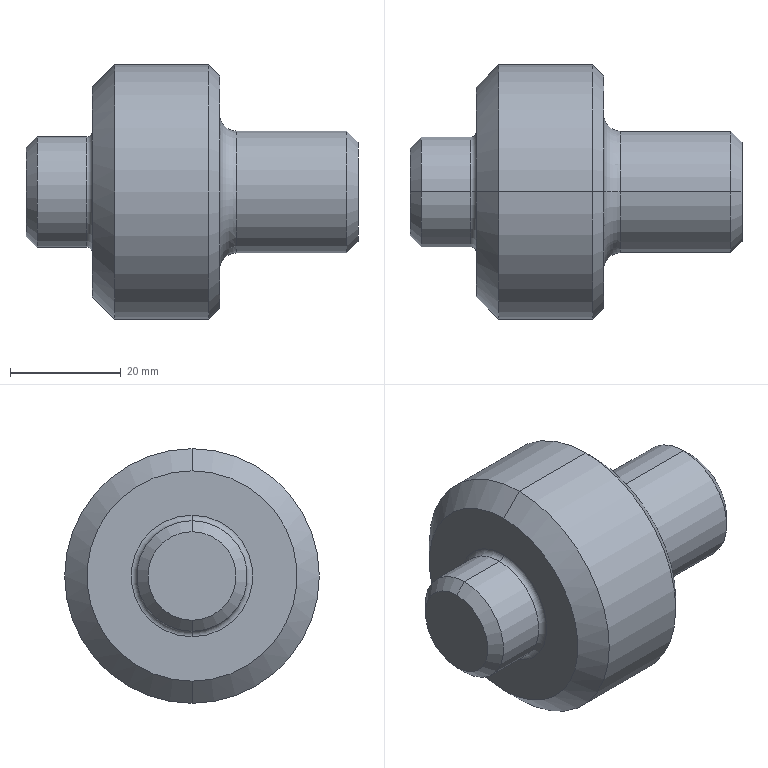Component | SolidWorks | THK-A1028TravelingMotorFlangeMountingAxis-1 | 1 solid | 26 faces | box 60 x 46 x 46 mm | volume 48569 mm3 | cone 10 | cylinder 8 | torus 4 | plane 4 | commonest cylinder face diameters 8.5 x2 22 x2 46 x2 20 x2 | material 45
build123d program:
from build123d import *

# Parameters (mm, degrees)
SKETCH1_R              = 10
BOSS_EXTRUDE1_DEPTH    = 6
SKETCH2_R              = 23
BOSS_EXTRUDE2_DEPTH    = 23
SKETCH3_R              = 11
BOSS_EXTRUDE3_DEPTH    = 25
M10_TAPPED_HOLE1_D     = 8.5
M10_TAPPED_HOLE1_DEPTH = 25
M10_TAPPED_HOLE1_TIP   = 2.554
CHAMFER1_SIZE          = 2
FILLET1_R              = 3
FILLET2_R              = 1
CHAMFER2_SIZE          = 4


with BuildPart() as part:
    # Sketch1 → Boss-Extrude1 (new, symmetric)
    with BuildSketch(Plane(origin=(0, 0, 0), x_dir=(0, 0, -1), z_dir=(1, 0, 0))):
        Circle(SKETCH1_R)
    extrude(amount=BOSS_EXTRUDE1_DEPTH, both=True)

    # Sketch2 → Boss-Extrude2 (add)
    with BuildSketch(Plane.ZY.offset(-6)):
        Circle(SKETCH2_R)
    extrude(amount=-BOSS_EXTRUDE2_DEPTH)

    # Sketch3 → Boss-Extrude3 (add)
    with BuildSketch(Plane.ZY.offset(-29)):
        Circle(SKETCH3_R)
    extrude(amount=-BOSS_EXTRUDE3_DEPTH)

    # M10 Tapped Hole1
    with Locations(Plane(origin=(54, 0, 0), x_dir=(0, 0, -1), z_dir=(1, 0, 0))):
        with Locations((0, 0)):
            Hole(M10_TAPPED_HOLE1_D / 2, depth=M10_TAPPED_HOLE1_DEPTH)
            with Locations((0, 0, -(M10_TAPPED_HOLE1_DEPTH + M10_TAPPED_HOLE1_TIP / 2))):  # 118° drill point
                Cone(0, M10_TAPPED_HOLE1_D / 2, M10_TAPPED_HOLE1_TIP, mode=Mode.SUBTRACT)

    # Chamfer1
    chamfer1_edges = [part.edges().sort_by_distance(p)[0] for p in [
        (54, 0, -11),
        (-6, 0, 10),
        (29, 0, -23),
    ]]
    chamfer(chamfer1_edges, length=CHAMFER1_SIZE)

    # Fillet1
    fillet1_edges = [part.edges().sort_by_distance(p)[0] for p in [
        (29, 0, -11),
    ]]
    fillet(fillet1_edges, radius=FILLET1_R)

    # Fillet2
    fillet2_edges = [part.edges().sort_by_distance(p)[0] for p in [
        (6, 0, 10),
    ]]
    fillet(fillet2_edges, radius=FILLET2_R)

    # Chamfer2
    chamfer2_edges = [part.edges().sort_by_distance(p)[0] for p in [
        (6, 0, -23),
    ]]
    chamfer(chamfer2_edges, length=CHAMFER2_SIZE)


solid = part.part

# Placed as in the assembly
solid = solid.moved(Location((79, 115, 321), (0, 0, 0)))
STEP:
#1=CARTESIAN_POINT('',(3.346,4.528,13.386));
#2=VERTEX_POINT('',#1);
#3=CARTESIAN_POINT('',(3.346,4.528,11.89));
#4=VERTEX_POINT('',#3);
#5=CARTESIAN_POINT('',(3.346,4.528,12.638));
#6=DIRECTION('',(-1.,0.,-0.));
#7=DIRECTION('',(0.,0.,1.));
#8=AXIS2_PLACEMENT_3D('',#5,#6,#7);
#9=CIRCLE('',#8,0.748);
#10=EDGE_CURVE('',#2,#4,#9,.T.);
#11=ORIENTED_EDGE('',*,*,#10,.F.);
#12=CARTESIAN_POINT('',(3.504,4.528,13.543));
#13=VERTEX_POINT('',#12);
#14=CARTESIAN_POINT('',(3.346,4.528,13.386));
#15=DIRECTION('',(0.7071,0.,0.7071));
#16=VECTOR('',#15,39.37);
#17=LINE('',#14,#16);
#18=EDGE_CURVE('',#2,#13,#17,.T.);
#19=ORIENTED_EDGE('',*,*,#18,.T.);
#20=CARTESIAN_POINT('',(3.504,4.528,11.732));
#21=VERTEX_POINT('',#20);
#22=CARTESIAN_POINT('',(3.504,4.528,12.638));
#23=DIRECTION('',(1.,0.,0.));
#24=DIRECTION('',(0.,0.,1.));
#25=AXIS2_PLACEMENT_3D('',#22,#23,#24);
#26=CIRCLE('',#25,0.9055);
#27=EDGE_CURVE('',#21,#13,#26,.T.);
#28=ORIENTED_EDGE('',*,*,#27,.F.);
#29=CARTESIAN_POINT('',(3.346,4.528,11.89));
#30=DIRECTION('',(0.7071,0.,-0.7071));
#31=VECTOR('',#30,39.37);
#32=LINE('',#29,#31);
#33=EDGE_CURVE('',#4,#21,#32,.T.);
#34=ORIENTED_EDGE('',*,*,#33,.F.);
#35=EDGE_LOOP('',(#11,#19,#28,#34));
#36=FACE_OUTER_BOUND('',#35,.T.);
#37=CARTESIAN_POINT('',(3.346,4.528,12.638));
#38=DIRECTION('',(1.,0.,0.));
#39=DIRECTION('',(0.,0.,-1.));
#40=AXIS2_PLACEMENT_3D('',#37,#38,#39);
#41=CONICAL_SURFACE('',#40,0.748,0.7854);
#42=ADVANCED_FACE('',(#36),#41,.T.);
#43=CARTESIAN_POINT('',(3.307,4.528,12.244));
#44=VERTEX_POINT('',#43);
#45=CARTESIAN_POINT('',(3.307,4.528,13.031));
#46=VERTEX_POINT('',#45);
#47=CARTESIAN_POINT('',(3.307,4.528,12.638));
#48=DIRECTION('',(-1.,0.,-0.));
#49=DIRECTION('',(0.,0.,1.));
#50=AXIS2_PLACEMENT_3D('',#47,#48,#49);
#51=CIRCLE('',#50,0.3937);
#52=EDGE_CURVE('',#44,#46,#51,.T.);
#53=ORIENTED_EDGE('',*,*,#52,.F.);
#54=CARTESIAN_POINT('',(3.346,4.528,12.205));
#55=VERTEX_POINT('',#54);
#56=CARTESIAN_POINT('',(3.307,4.528,12.205));
#57=DIRECTION('',(-0.,1.,0.));
#58=DIRECTION('',(0.,0.,1.));
#59=AXIS2_PLACEMENT_3D('',#56,#57,#58);
#60=CIRCLE('',#59,0.03937);
#61=EDGE_CURVE('',#44,#55,#60,.T.);
#62=ORIENTED_EDGE('',*,*,#61,.T.);
#63=CARTESIAN_POINT('',(3.346,4.528,13.071));
#64=VERTEX_POINT('',#63);
#65=CARTESIAN_POINT('',(3.346,4.528,12.638));
#66=DIRECTION('',(1.,0.,0.));
#67=DIRECTION('',(0.,0.,1.));
#68=AXIS2_PLACEMENT_3D('',#65,#66,#67);
#69=CIRCLE('',#68,0.4331);
#70=EDGE_CURVE('',#64,#55,#69,.T.);
#71=ORIENTED_EDGE('',*,*,#70,.F.);
#72=CARTESIAN_POINT('',(3.307,4.528,13.071));
#73=DIRECTION('',(0.,-1.,0.));
#74=DIRECTION('',(0.,0.,-1.));
#75=AXIS2_PLACEMENT_3D('',#72,#73,#74);
#76=CIRCLE('',#75,0.03937);
#77=EDGE_CURVE('',#46,#64,#76,.T.);
#78=ORIENTED_EDGE('',*,*,#77,.F.);
#79=EDGE_LOOP('',(#53,#62,#71,#78));
#80=FACE_OUTER_BOUND('',#79,.T.);
#81=CARTESIAN_POINT('',(3.307,4.528,12.638));
#82=DIRECTION('',(-1.,0.,-0.));
#83=DIRECTION('',(-0.,0.,1.));
#84=AXIS2_PLACEMENT_3D('',#81,#82,#83);
#85=TOROIDAL_SURFACE('',#84,0.4331,0.03937);
#86=ADVANCED_FACE('',(#80),#85,.F.);
#87=CARTESIAN_POINT('',(4.252,4.528,12.087));
#88=VERTEX_POINT('',#87);
#89=CARTESIAN_POINT('',(4.252,4.528,13.189));
#90=VERTEX_POINT('',#89);
#91=CARTESIAN_POINT('',(4.252,4.528,12.638));
#92=DIRECTION('',(-1.,0.,-0.));
#93=DIRECTION('',(0.,0.,1.));
#94=AXIS2_PLACEMENT_3D('',#91,#92,#93);
#95=CIRCLE('',#94,0.5512);
#96=EDGE_CURVE('',#88,#90,#95,.T.);
#97=ORIENTED_EDGE('',*,*,#96,.F.);
#98=CARTESIAN_POINT('',(4.37,4.528,12.205));
#99=VERTEX_POINT('',#98);
#100=CARTESIAN_POINT('',(4.37,4.528,12.087));
#101=DIRECTION('',(-0.,1.,0.));
#102=DIRECTION('',(0.,0.,1.));
#103=AXIS2_PLACEMENT_3D('',#100,#101,#102);
#104=CIRCLE('',#103,0.1181);
#105=EDGE_CURVE('',#88,#99,#104,.T.);
#106=ORIENTED_EDGE('',*,*,#105,.T.);
#107=CARTESIAN_POINT('',(4.37,4.528,13.071));
#108=VERTEX_POINT('',#107);
#109=CARTESIAN_POINT('',(4.37,4.528,12.638));
#110=DIRECTION('',(1.,0.,0.));
#111=DIRECTION('',(0.,0.,1.));
#112=AXIS2_PLACEMENT_3D('',#109,#110,#111);
#113=CIRCLE('',#112,0.4331);
#114=EDGE_CURVE('',#108,#99,#113,.T.);
#115=ORIENTED_EDGE('',*,*,#114,.F.);
#116=CARTESIAN_POINT('',(4.37,4.528,13.189));
#117=DIRECTION('',(0.,-1.,0.));
#118=DIRECTION('',(0.,0.,-1.));
#119=AXIS2_PLACEMENT_3D('',#116,#117,#118);
#120=CIRCLE('',#119,0.1181);
#121=EDGE_CURVE('',#90,#108,#120,.T.);
#122=ORIENTED_EDGE('',*,*,#121,.F.);
#123=EDGE_LOOP('',(#97,#106,#115,#122));
#124=FACE_OUTER_BOUND('',#123,.T.);
#125=CARTESIAN_POINT('',(4.37,4.528,12.638));
#126=DIRECTION('',(-1.,0.,-0.));
#127=DIRECTION('',(-0.,0.,1.));
#128=AXIS2_PLACEMENT_3D('',#125,#126,#127);
#129=TOROIDAL_SURFACE('',#128,0.5512,0.1181);
#130=ADVANCED_FACE('',(#124),#129,.F.);
#131=CARTESIAN_POINT('',(4.252,4.528,11.811));
#132=VERTEX_POINT('',#131);
#133=CARTESIAN_POINT('',(4.252,4.528,13.465));
#134=VERTEX_POINT('',#133);
#135=CARTESIAN_POINT('',(4.252,4.528,12.638));
#136=DIRECTION('',(1.,0.,0.));
#137=DIRECTION('',(0.,0.,1.));
#138=AXIS2_PLACEMENT_3D('',#135,#136,#137);
#139=CIRCLE('',#138,0.8268);
#140=EDGE_CURVE('',#132,#134,#139,.T.);
#141=ORIENTED_EDGE('',*,*,#140,.F.);
#142=CARTESIAN_POINT('',(4.173,4.528,11.732));
#143=VERTEX_POINT('',#142);
#144=CARTESIAN_POINT('',(4.173,4.528,11.732));
#145=DIRECTION('',(-0.7071,0.,-0.7071));
#146=VECTOR('',#145,39.37);
#147=LINE('',#144,#146);
#148=EDGE_CURVE('',#132,#143,#147,.T.);
#149=ORIENTED_EDGE('',*,*,#148,.T.);
#150=CARTESIAN_POINT('',(4.173,4.528,13.543));
#151=VERTEX_POINT('',#150);
#152=CARTESIAN_POINT('',(4.173,4.528,12.638));
#153=DIRECTION('',(-1.,0.,-0.));
#154=DIRECTION('',(0.,0.,1.));
#155=AXIS2_PLACEMENT_3D('',#152,#153,#154);
#156=CIRCLE('',#155,0.9055);
#157=EDGE_CURVE('',#151,#143,#156,.T.);
#158=ORIENTED_EDGE('',*,*,#157,.F.);
#159=CARTESIAN_POINT('',(4.173,4.528,13.543));
#160=DIRECTION('',(-0.7071,0.,0.7071));
#161=VECTOR('',#160,39.37);
#162=LINE('',#159,#161);
#163=EDGE_CURVE('',#134,#151,#162,.T.);
#164=ORIENTED_EDGE('',*,*,#163,.F.);
#165=EDGE_LOOP('',(#141,#149,#158,#164));
#166=FACE_OUTER_BOUND('',#165,.T.);
#167=CARTESIAN_POINT('',(4.173,4.528,12.638));
#168=DIRECTION('',(-1.,0.,-0.));
#169=DIRECTION('',(0.,0.,1.));
#170=AXIS2_PLACEMENT_3D('',#167,#168,#169);
#171=CONICAL_SURFACE('',#170,0.9055,0.7854);
#172=ADVANCED_FACE('',(#166),#171,.T.);
#173=CARTESIAN_POINT('',(5.236,4.528,12.283));
#174=VERTEX_POINT('',#173);
#175=CARTESIAN_POINT('',(5.236,4.528,12.992));
#176=VERTEX_POINT('',#175);
#177=CARTESIAN_POINT('',(5.236,4.528,12.638));
#178=DIRECTION('',(1.,0.,0.));
#179=DIRECTION('',(0.,0.,1.));
#180=AXIS2_PLACEMENT_3D('',#177,#178,#179);
#181=CIRCLE('',#180,0.3543);
#182=EDGE_CURVE('',#174,#176,#181,.T.);
#183=ORIENTED_EDGE('',*,*,#182,.F.);
#184=CARTESIAN_POINT('',(5.157,4.528,12.205));
#185=VERTEX_POINT('',#184);
#186=CARTESIAN_POINT('',(5.157,4.528,12.205));
#187=DIRECTION('',(-0.7071,0.,-0.7071));
#188=VECTOR('',#187,39.37);
#189=LINE('',#186,#188);
#190=EDGE_CURVE('',#174,#185,#189,.T.);
#191=ORIENTED_EDGE('',*,*,#190,.T.);
#192=CARTESIAN_POINT('',(5.157,4.528,13.071));
#193=VERTEX_POINT('',#192);
#194=CARTESIAN_POINT('',(5.157,4.528,12.638));
#195=DIRECTION('',(-1.,0.,-0.));
#196=DIRECTION('',(0.,0.,1.));
#197=AXIS2_PLACEMENT_3D('',#194,#195,#196);
#198=CIRCLE('',#197,0.4331);
#199=EDGE_CURVE('',#193,#185,#198,.T.);
#200=ORIENTED_EDGE('',*,*,#199,.F.);
#201=CARTESIAN_POINT('',(5.157,4.528,13.071));
#202=DIRECTION('',(-0.7071,0.,0.7071));
#203=VECTOR('',#202,39.37);
#204=LINE('',#201,#203);
#205=EDGE_CURVE('',#176,#193,#204,.T.);
#206=ORIENTED_EDGE('',*,*,#205,.F.);
#207=EDGE_LOOP('',(#183,#191,#200,#206));
#208=FACE_OUTER_BOUND('',#207,.T.);
#209=CARTESIAN_POINT('',(5.157,4.528,12.638));
#210=DIRECTION('',(-1.,0.,-0.));
#211=DIRECTION('',(0.,0.,1.));
#212=AXIS2_PLACEMENT_3D('',#209,#210,#211);
#213=CONICAL_SURFACE('',#212,0.4331,0.7854);
#214=ADVANCED_FACE('',(#208),#213,.T.);
#215=CARTESIAN_POINT('',(2.874,4.528,12.953));
#216=VERTEX_POINT('',#215);
#217=CARTESIAN_POINT('',(2.874,4.528,12.323));
#218=VERTEX_POINT('',#217);
#219=CARTESIAN_POINT('',(2.874,4.528,12.638));
#220=DIRECTION('',(-1.,0.,0.));
#221=DIRECTION('',(0.,0.,-1.));
#222=AXIS2_PLACEMENT_3D('',#219,#220,#221);
#223=CIRCLE('',#222,0.315);
#224=EDGE_CURVE('',#216,#218,#223,.T.);
#225=ORIENTED_EDGE('',*,*,#224,.F.);
#226=CARTESIAN_POINT('',(2.953,4.528,13.031));
#227=VERTEX_POINT('',#226);
#228=CARTESIAN_POINT('',(2.953,4.528,13.031));
#229=DIRECTION('',(0.7071,0.,0.7071));
#230=VECTOR('',#229,39.37);
#231=LINE('',#228,#230);
#232=EDGE_CURVE('',#216,#227,#231,.T.);
#233=ORIENTED_EDGE('',*,*,#232,.T.);
#234=CARTESIAN_POINT('',(2.953,4.528,12.244));
#235=VERTEX_POINT('',#234);
#236=CARTESIAN_POINT('',(2.953,4.528,12.638));
#237=DIRECTION('',(1.,0.,0.));
#238=DIRECTION('',(0.,0.,-1.));
#239=AXIS2_PLACEMENT_3D('',#236,#237,#238);
#240=CIRCLE('',#239,0.3937);
#241=EDGE_CURVE('',#235,#227,#240,.T.);
#242=ORIENTED_EDGE('',*,*,#241,.F.);
#243=CARTESIAN_POINT('',(2.953,4.528,12.244));
#244=DIRECTION('',(0.7071,0.,-0.7071));
#245=VECTOR('',#244,39.37);
#246=LINE('',#243,#245);
#247=EDGE_CURVE('',#218,#235,#246,.T.);
#248=ORIENTED_EDGE('',*,*,#247,.F.);
#249=EDGE_LOOP('',(#225,#233,#242,#248));
#250=FACE_OUTER_BOUND('',#249,.T.);
#251=CARTESIAN_POINT('',(2.953,4.528,12.638));
#252=DIRECTION('',(1.,0.,0.));
#253=DIRECTION('',(0.,0.,-1.));
#254=AXIS2_PLACEMENT_3D('',#251,#252,#253);
#255=CONICAL_SURFACE('',#254,0.3937,0.7854);
#256=ADVANCED_FACE('',(#250),#255,.T.);
#257=CARTESIAN_POINT('',(4.252,4.528,12.805));
#258=VERTEX_POINT('',#257);
#259=CARTESIAN_POINT('',(4.252,4.528,12.47));
#260=VERTEX_POINT('',#259);
#261=CARTESIAN_POINT('',(4.252,4.528,12.638));
#262=DIRECTION('',(1.,0.,0.));
#263=DIRECTION('',(0.,0.,-1.));
#264=AXIS2_PLACEMENT_3D('',#261,#262,#263);
#265=CIRCLE('',#264,0.1673);
#266=EDGE_CURVE('',#258,#260,#265,.T.);
#267=ORIENTED_EDGE('',*,*,#266,.F.);
#268=CARTESIAN_POINT('',(5.236,4.528,12.805));
#269=VERTEX_POINT('',#268);
#270=CARTESIAN_POINT('',(5.236,4.528,12.805));
#271=DIRECTION('',(1.,0.,0.));
#272=VECTOR('',#271,39.37);
#273=LINE('',#270,#272);
#274=EDGE_CURVE('',#258,#269,#273,.T.);
#275=ORIENTED_EDGE('',*,*,#274,.T.);
#276=CARTESIAN_POINT('',(5.236,4.528,12.47));
#277=VERTEX_POINT('',#276);
#278=CARTESIAN_POINT('',(5.236,4.528,12.638));
#279=DIRECTION('',(1.,0.,0.));
#280=DIRECTION('',(0.,0.,-1.));
#281=AXIS2_PLACEMENT_3D('',#278,#279,#280);
#282=CIRCLE('',#281,0.1673);
#283=EDGE_CURVE('',#269,#277,#282,.T.);
#284=ORIENTED_EDGE('',*,*,#283,.T.);
#285=CARTESIAN_POINT('',(5.236,4.528,12.47));
#286=DIRECTION('',(1.,0.,0.));
#287=VECTOR('',#286,39.37);
#288=LINE('',#285,#287);
#289=EDGE_CURVE('',#260,#277,#288,.T.);
#290=ORIENTED_EDGE('',*,*,#289,.F.);
#291=EDGE_LOOP('',(#267,#275,#284,#290));
#292=FACE_OUTER_BOUND('',#291,.T.);
#293=CARTESIAN_POINT('',(5.236,4.528,12.638));
#294=DIRECTION('',(1.,0.,0.));
#295=DIRECTION('',(0.,0.,-1.));
#296=AXIS2_PLACEMENT_3D('',#293,#294,#295);
#297=CYLINDRICAL_SURFACE('',#296,0.1673);
#298=ADVANCED_FACE('',(#292),#297,.F.);
#299=CARTESIAN_POINT('',(4.151,4.528,12.638));
#300=VERTEX_POINT('',#299);
#301=CARTESIAN_POINT('',(4.252,4.528,12.47));
#302=DIRECTION('',(0.515,0.,-0.8572));
#303=VECTOR('',#302,39.37);
#304=LINE('',#301,#303);
#305=EDGE_CURVE('',#300,#260,#304,.T.);
#306=ORIENTED_EDGE('',*,*,#305,.F.);
#307=CARTESIAN_POINT('',(4.252,4.528,12.805));
#308=DIRECTION('',(0.515,0.,0.8572));
#309=VECTOR('',#308,39.37);
#310=LINE('',#307,#309);
#311=EDGE_CURVE('',#300,#258,#310,.T.);
#312=ORIENTED_EDGE('',*,*,#311,.T.);
#313=ORIENTED_EDGE('',*,*,#266,.T.);
#314=EDGE_LOOP('',(#306,#312,#313));
#315=FACE_OUTER_BOUND('',#314,.T.);
#316=CARTESIAN_POINT('',(4.252,4.528,12.638));
#317=DIRECTION('',(1.,0.,0.));
#318=DIRECTION('',(0.,0.,-1.));
#319=AXIS2_PLACEMENT_3D('',#316,#317,#318);
#320=CONICAL_SURFACE('',#319,0.1673,1.03);
#321=ADVANCED_FACE('',(#315),#320,.F.);
#322=ORIENTED_EDGE('',*,*,#199,.T.);
#323=CARTESIAN_POINT('',(5.236,4.528,12.205));
#324=DIRECTION('',(-1.,0.,-0.));
#325=VECTOR('',#324,39.37);
#326=LINE('',#323,#325);
#327=EDGE_CURVE('',#185,#99,#326,.T.);
#328=ORIENTED_EDGE('',*,*,#327,.T.);
#329=CARTESIAN_POINT('',(4.37,4.528,12.638));
#330=DIRECTION('',(1.,0.,0.));
#331=DIRECTION('',(0.,0.,1.));
#332=AXIS2_PLACEMENT_3D('',#329,#330,#331);
#333=CIRCLE('',#332,0.4331);
#334=EDGE_CURVE('',#99,#108,#333,.T.);
#335=ORIENTED_EDGE('',*,*,#334,.T.);
#336=CARTESIAN_POINT('',(5.236,4.528,13.071));
#337=DIRECTION('',(-1.,0.,-0.));
#338=VECTOR('',#337,39.37);
#339=LINE('',#336,#338);
#340=EDGE_CURVE('',#193,#108,#339,.T.);
#341=ORIENTED_EDGE('',*,*,#340,.F.);
#342=EDGE_LOOP('',(#322,#328,#335,#341));
#343=FACE_OUTER_BOUND('',#342,.T.);
#344=CARTESIAN_POINT('',(5.236,4.528,12.638));
#345=DIRECTION('',(-1.,0.,-0.));
#346=DIRECTION('',(0.,0.,1.));
#347=AXIS2_PLACEMENT_3D('',#344,#345,#346);
#348=CYLINDRICAL_SURFACE('',#347,0.4331);
#349=ADVANCED_FACE('',(#343),#348,.T.);
#350=ORIENTED_EDGE('',*,*,#157,.T.);
#351=CARTESIAN_POINT('',(4.252,4.528,11.732));
#352=DIRECTION('',(-1.,0.,-0.));
#353=VECTOR('',#352,39.37);
#354=LINE('',#351,#353);
#355=EDGE_CURVE('',#143,#21,#354,.T.);
#356=ORIENTED_EDGE('',*,*,#355,.T.);
#357=ORIENTED_EDGE('',*,*,#27,.T.);
#358=CARTESIAN_POINT('',(4.252,4.528,13.543));
#359=DIRECTION('',(-1.,0.,-0.));
#360=VECTOR('',#359,39.37);
#361=LINE('',#358,#360);
#362=EDGE_CURVE('',#151,#13,#361,.T.);
#363=ORIENTED_EDGE('',*,*,#362,.F.);
#364=EDGE_LOOP('',(#350,#356,#357,#363));
#365=FACE_OUTER_BOUND('',#364,.T.);
#366=CARTESIAN_POINT('',(4.252,4.528,12.638));
#367=DIRECTION('',(-1.,0.,-0.));
#368=DIRECTION('',(0.,0.,1.));
#369=AXIS2_PLACEMENT_3D('',#366,#367,#368);
#370=CYLINDRICAL_SURFACE('',#369,0.9055);
#371=ADVANCED_FACE('',(#365),#370,.T.);
#372=CARTESIAN_POINT('',(3.307,4.528,12.638));
#373=DIRECTION('',(-1.,0.,-0.));
#374=DIRECTION('',(0.,0.,1.));
#375=AXIS2_PLACEMENT_3D('',#372,#373,#374);
#376=CIRCLE('',#375,0.3937);
#377=EDGE_CURVE('',#46,#44,#376,.T.);
#378=ORIENTED_EDGE('',*,*,#377,.T.);
#379=CARTESIAN_POINT('',(3.346,4.528,12.244));
#380=DIRECTION('',(-1.,0.,0.));
#381=VECTOR('',#380,39.37);
#382=LINE('',#379,#381);
#383=EDGE_CURVE('',#44,#235,#382,.T.);
#384=ORIENTED_EDGE('',*,*,#383,.T.);
#385=ORIENTED_EDGE('',*,*,#241,.T.);
#386=CARTESIAN_POINT('',(3.346,4.528,13.031));
#387=DIRECTION('',(-1.,0.,0.));
#388=VECTOR('',#387,39.37);
#389=LINE('',#386,#388);
#390=EDGE_CURVE('',#46,#227,#389,.T.);
#391=ORIENTED_EDGE('',*,*,#390,.F.);
#392=EDGE_LOOP('',(#378,#384,#385,#391));
#393=FACE_OUTER_BOUND('',#392,.T.);
#394=CARTESIAN_POINT('',(3.346,4.528,12.638));
#395=DIRECTION('',(-1.,0.,0.));
#396=DIRECTION('',(0.,0.,1.));
#397=AXIS2_PLACEMENT_3D('',#394,#395,#396);
#398=CYLINDRICAL_SURFACE('',#397,0.3937);
#399=ADVANCED_FACE('',(#393),#398,.T.);
#400=ORIENTED_EDGE('',*,*,#383,.F.);
#401=ORIENTED_EDGE('',*,*,#52,.T.);
#402=ORIENTED_EDGE('',*,*,#390,.T.);
#403=CARTESIAN_POINT('',(2.953,4.528,12.638));
#404=DIRECTION('',(1.,0.,0.));
#405=DIRECTION('',(0.,0.,-1.));
#406=AXIS2_PLACEMENT_3D('',#403,#404,#405);
#407=CIRCLE('',#406,0.3937);
#408=EDGE_CURVE('',#227,#235,#407,.T.);
#409=ORIENTED_EDGE('',*,*,#408,.T.);
#410=EDGE_LOOP('',(#400,#401,#402,#409));
#411=FACE_OUTER_BOUND('',#410,.T.);
#412=CARTESIAN_POINT('',(3.346,4.528,12.638));
#413=DIRECTION('',(-1.,0.,0.));
#414=DIRECTION('',(0.,0.,1.));
#415=AXIS2_PLACEMENT_3D('',#412,#413,#414);
#416=CYLINDRICAL_SURFACE('',#415,0.3937);
#417=ADVANCED_FACE('',(#411),#416,.T.);
#418=CARTESIAN_POINT('',(2.874,4.528,12.638));
#419=DIRECTION('',(-1.,0.,0.));
#420=DIRECTION('',(0.,0.,-1.));
#421=AXIS2_PLACEMENT_3D('',#418,#419,#420);
#422=CIRCLE('',#421,0.315);
#423=EDGE_CURVE('',#218,#216,#422,.T.);
#424=ORIENTED_EDGE('',*,*,#423,.T.);
#425=ORIENTED_EDGE('',*,*,#224,.T.);
#426=EDGE_LOOP('',(#424,#425));
#427=FACE_OUTER_BOUND('',#426,.T.);
#428=CARTESIAN_POINT('',(2.874,4.528,12.638));
#429=DIRECTION('',(1.,0.,0.));
#430=DIRECTION('',(0.,0.,-1.));
#431=AXIS2_PLACEMENT_3D('',#428,#429,#430);
#432=PLANE('',#431);
#433=ADVANCED_FACE('',(#427),#432,.F.);
#434=CARTESIAN_POINT('',(3.346,4.528,12.638));
#435=DIRECTION('',(-1.,0.,-0.));
#436=DIRECTION('',(0.,0.,1.));
#437=AXIS2_PLACEMENT_3D('',#434,#435,#436);
#438=CIRCLE('',#437,0.748);
#439=EDGE_CURVE('',#4,#2,#438,.T.);
#440=ORIENTED_EDGE('',*,*,#439,.T.);
#441=ORIENTED_EDGE('',*,*,#10,.T.);
#442=EDGE_LOOP('',(#440,#441));
#443=FACE_OUTER_BOUND('',#442,.T.);
#444=ORIENTED_EDGE('',*,*,#70,.T.);
#445=CARTESIAN_POINT('',(3.346,4.528,12.638));
#446=DIRECTION('',(1.,0.,0.));
#447=DIRECTION('',(0.,0.,1.));
#448=AXIS2_PLACEMENT_3D('',#445,#446,#447);
#449=CIRCLE('',#448,0.4331);
#450=EDGE_CURVE('',#55,#64,#449,.T.);
#451=ORIENTED_EDGE('',*,*,#450,.T.);
#452=EDGE_LOOP('',(#444,#451));
#453=FACE_BOUND('',#452,.T.);
#454=CARTESIAN_POINT('',(3.346,4.528,12.638));
#455=DIRECTION('',(-1.,0.,-0.));
#456=DIRECTION('',(-0.,0.,1.));
#457=AXIS2_PLACEMENT_3D('',#454,#455,#456);
#458=PLANE('',#457);
#459=ADVANCED_FACE('',(#443,#453),#458,.T.);
#460=ORIENTED_EDGE('',*,*,#355,.F.);
#461=CARTESIAN_POINT('',(4.173,4.528,12.638));
#462=DIRECTION('',(-1.,0.,-0.));
#463=DIRECTION('',(0.,0.,1.));
#464=AXIS2_PLACEMENT_3D('',#461,#462,#463);
#465=CIRCLE('',#464,0.9055);
#466=EDGE_CURVE('',#143,#151,#465,.T.);
#467=ORIENTED_EDGE('',*,*,#466,.T.);
#468=ORIENTED_EDGE('',*,*,#362,.T.);
#469=CARTESIAN_POINT('',(3.504,4.528,12.638));
#470=DIRECTION('',(1.,0.,0.));
#471=DIRECTION('',(0.,0.,1.));
#472=AXIS2_PLACEMENT_3D('',#469,#470,#471);
#473=CIRCLE('',#472,0.9055);
#474=EDGE_CURVE('',#13,#21,#473,.T.);
#475=ORIENTED_EDGE('',*,*,#474,.T.);
#476=EDGE_LOOP('',(#460,#467,#468,#475));
#477=FACE_OUTER_BOUND('',#476,.T.);
#478=CARTESIAN_POINT('',(4.252,4.528,12.638));
#479=DIRECTION('',(-1.,0.,-0.));
#480=DIRECTION('',(0.,0.,1.));
#481=AXIS2_PLACEMENT_3D('',#478,#479,#480);
#482=CYLINDRICAL_SURFACE('',#481,0.9055);
#483=ADVANCED_FACE('',(#477),#482,.T.);
#484=CARTESIAN_POINT('',(4.252,4.528,12.638));
#485=DIRECTION('',(-1.,0.,-0.));
#486=DIRECTION('',(0.,0.,1.));
#487=AXIS2_PLACEMENT_3D('',#484,#485,#486);
#488=CIRCLE('',#487,0.5512);
#489=EDGE_CURVE('',#90,#88,#488,.T.);
#490=ORIENTED_EDGE('',*,*,#489,.T.);
#491=ORIENTED_EDGE('',*,*,#96,.T.);
#492=EDGE_LOOP('',(#490,#491));
#493=FACE_BOUND('',#492,.T.);
#494=CARTESIAN_POINT('',(4.252,4.528,12.638));
#495=DIRECTION('',(1.,0.,0.));
#496=DIRECTION('',(0.,0.,1.));
#497=AXIS2_PLACEMENT_3D('',#494,#495,#496);
#498=CIRCLE('',#497,0.8268);
#499=EDGE_CURVE('',#134,#132,#498,.T.);
#500=ORIENTED_EDGE('',*,*,#499,.T.);
#501=ORIENTED_EDGE('',*,*,#140,.T.);
#502=EDGE_LOOP('',(#500,#501));
#503=FACE_OUTER_BOUND('',#502,.T.);
#504=CARTESIAN_POINT('',(4.252,4.528,12.638));
#505=DIRECTION('',(-1.,0.,-0.));
#506=DIRECTION('',(-0.,0.,1.));
#507=AXIS2_PLACEMENT_3D('',#504,#505,#506);
#508=PLANE('',#507);
#509=ADVANCED_FACE('',(#493,#503),#508,.F.);
#510=ORIENTED_EDGE('',*,*,#327,.F.);
#511=CARTESIAN_POINT('',(5.157,4.528,12.638));
#512=DIRECTION('',(-1.,0.,-0.));
#513=DIRECTION('',(0.,0.,1.));
#514=AXIS2_PLACEMENT_3D('',#511,#512,#513);
#515=CIRCLE('',#514,0.4331);
#516=EDGE_CURVE('',#185,#193,#515,.T.);
#517=ORIENTED_EDGE('',*,*,#516,.T.);
#518=ORIENTED_EDGE('',*,*,#340,.T.);
#519=ORIENTED_EDGE('',*,*,#114,.T.);
#520=EDGE_LOOP('',(#510,#517,#518,#519));
#521=FACE_OUTER_BOUND('',#520,.T.);
#522=CARTESIAN_POINT('',(5.236,4.528,12.638));
#523=DIRECTION('',(-1.,0.,-0.));
#524=DIRECTION('',(0.,0.,1.));
#525=AXIS2_PLACEMENT_3D('',#522,#523,#524);
#526=CYLINDRICAL_SURFACE('',#525,0.4331);
#527=ADVANCED_FACE('',(#521),#526,.T.);
#528=CARTESIAN_POINT('',(5.236,4.528,12.638));
#529=DIRECTION('',(1.,0.,0.));
#530=DIRECTION('',(0.,0.,1.));
#531=AXIS2_PLACEMENT_3D('',#528,#529,#530);
#532=CIRCLE('',#531,0.3543);
#533=EDGE_CURVE('',#176,#174,#532,.T.);
#534=ORIENTED_EDGE('',*,*,#533,.T.);
#535=ORIENTED_EDGE('',*,*,#182,.T.);
#536=EDGE_LOOP('',(#534,#535));
#537=FACE_OUTER_BOUND('',#536,.T.);
#538=CARTESIAN_POINT('',(5.236,4.528,12.638));
#539=DIRECTION('',(1.,0.,0.));
#540=DIRECTION('',(0.,0.,-1.));
#541=AXIS2_PLACEMENT_3D('',#538,#539,#540);
#542=CIRCLE('',#541,0.1673);
#543=EDGE_CURVE('',#277,#269,#542,.T.);
#544=ORIENTED_EDGE('',*,*,#543,.F.);
#545=ORIENTED_EDGE('',*,*,#283,.F.);
#546=EDGE_LOOP('',(#544,#545));
#547=FACE_BOUND('',#546,.T.);
#548=CARTESIAN_POINT('',(5.236,4.528,12.638));
#549=DIRECTION('',(-1.,0.,-0.));
#550=DIRECTION('',(-0.,0.,1.));
#551=AXIS2_PLACEMENT_3D('',#548,#549,#550);
#552=PLANE('',#551);
#553=ADVANCED_FACE('',(#537,#547),#552,.F.);
#554=ORIENTED_EDGE('',*,*,#311,.F.);
#555=ORIENTED_EDGE('',*,*,#305,.T.);
#556=CARTESIAN_POINT('',(4.252,4.528,12.638));
#557=DIRECTION('',(1.,0.,0.));
#558=DIRECTION('',(0.,0.,-1.));
#559=AXIS2_PLACEMENT_3D('',#556,#557,#558);
#560=CIRCLE('',#559,0.1673);
#561=EDGE_CURVE('',#260,#258,#560,.T.);
#562=ORIENTED_EDGE('',*,*,#561,.T.);
#563=EDGE_LOOP('',(#554,#555,#562));
#564=FACE_OUTER_BOUND('',#563,.T.);
#565=CARTESIAN_POINT('',(4.252,4.528,12.638));
#566=DIRECTION('',(1.,0.,0.));
#567=DIRECTION('',(0.,0.,-1.));
#568=AXIS2_PLACEMENT_3D('',#565,#566,#567);
#569=CONICAL_SURFACE('',#568,0.1673,1.03);
#570=ADVANCED_FACE('',(#564),#569,.F.);
#571=ORIENTED_EDGE('',*,*,#274,.F.);
#572=ORIENTED_EDGE('',*,*,#561,.F.);
#573=ORIENTED_EDGE('',*,*,#289,.T.);
#574=ORIENTED_EDGE('',*,*,#543,.T.);
#575=EDGE_LOOP('',(#571,#572,#573,#574));
#576=FACE_OUTER_BOUND('',#575,.T.);
#577=CARTESIAN_POINT('',(5.236,4.528,12.638));
#578=DIRECTION('',(1.,0.,0.));
#579=DIRECTION('',(0.,0.,-1.));
#580=AXIS2_PLACEMENT_3D('',#577,#578,#579);
#581=CYLINDRICAL_SURFACE('',#580,0.1673);
#582=ADVANCED_FACE('',(#576),#581,.F.);
#583=ORIENTED_EDGE('',*,*,#232,.F.);
#584=ORIENTED_EDGE('',*,*,#423,.F.);
#585=ORIENTED_EDGE('',*,*,#247,.T.);
#586=ORIENTED_EDGE('',*,*,#408,.F.);
#587=EDGE_LOOP('',(#583,#584,#585,#586));
#588=FACE_OUTER_BOUND('',#587,.T.);
#589=CARTESIAN_POINT('',(2.953,4.528,12.638));
#590=DIRECTION('',(1.,0.,0.));
#591=DIRECTION('',(0.,0.,-1.));
#592=AXIS2_PLACEMENT_3D('',#589,#590,#591);
#593=CONICAL_SURFACE('',#592,0.3937,0.7854);
#594=ADVANCED_FACE('',(#588),#593,.T.);
#595=ORIENTED_EDGE('',*,*,#190,.F.);
#596=ORIENTED_EDGE('',*,*,#533,.F.);
#597=ORIENTED_EDGE('',*,*,#205,.T.);
#598=ORIENTED_EDGE('',*,*,#516,.F.);
#599=EDGE_LOOP('',(#595,#596,#597,#598));
#600=FACE_OUTER_BOUND('',#599,.T.);
#601=CARTESIAN_POINT('',(5.157,4.528,12.638));
#602=DIRECTION('',(-1.,0.,-0.));
#603=DIRECTION('',(0.,0.,1.));
#604=AXIS2_PLACEMENT_3D('',#601,#602,#603);
#605=CONICAL_SURFACE('',#604,0.4331,0.7854);
#606=ADVANCED_FACE('',(#600),#605,.T.);
#607=ORIENTED_EDGE('',*,*,#148,.F.);
#608=ORIENTED_EDGE('',*,*,#499,.F.);
#609=ORIENTED_EDGE('',*,*,#163,.T.);
#610=ORIENTED_EDGE('',*,*,#466,.F.);
#611=EDGE_LOOP('',(#607,#608,#609,#610));
#612=FACE_OUTER_BOUND('',#611,.T.);
#613=CARTESIAN_POINT('',(4.173,4.528,12.638));
#614=DIRECTION('',(-1.,0.,-0.));
#615=DIRECTION('',(0.,0.,1.));
#616=AXIS2_PLACEMENT_3D('',#613,#614,#615);
#617=CONICAL_SURFACE('',#616,0.9055,0.7854);
#618=ADVANCED_FACE('',(#612),#617,.T.);
#619=ORIENTED_EDGE('',*,*,#105,.F.);
#620=ORIENTED_EDGE('',*,*,#489,.F.);
#621=ORIENTED_EDGE('',*,*,#121,.T.);
#622=ORIENTED_EDGE('',*,*,#334,.F.);
#623=EDGE_LOOP('',(#619,#620,#621,#622));
#624=FACE_OUTER_BOUND('',#623,.T.);
#625=CARTESIAN_POINT('',(4.37,4.528,12.638));
#626=DIRECTION('',(-1.,0.,-0.));
#627=DIRECTION('',(-0.,0.,1.));
#628=AXIS2_PLACEMENT_3D('',#625,#626,#627);
#629=TOROIDAL_SURFACE('',#628,0.5512,0.1181);
#630=ADVANCED_FACE('',(#624),#629,.F.);
#631=ORIENTED_EDGE('',*,*,#61,.F.);
#632=ORIENTED_EDGE('',*,*,#377,.F.);
#633=ORIENTED_EDGE('',*,*,#77,.T.);
#634=ORIENTED_EDGE('',*,*,#450,.F.);
#635=EDGE_LOOP('',(#631,#632,#633,#634));
#636=FACE_OUTER_BOUND('',#635,.T.);
#637=CARTESIAN_POINT('',(3.307,4.528,12.638));
#638=DIRECTION('',(-1.,0.,-0.));
#639=DIRECTION('',(-0.,0.,1.));
#640=AXIS2_PLACEMENT_3D('',#637,#638,#639);
#641=TOROIDAL_SURFACE('',#640,0.4331,0.03937);
#642=ADVANCED_FACE('',(#636),#641,.F.);
#643=ORIENTED_EDGE('',*,*,#18,.F.);
#644=ORIENTED_EDGE('',*,*,#439,.F.);
#645=ORIENTED_EDGE('',*,*,#33,.T.);
#646=ORIENTED_EDGE('',*,*,#474,.F.);
#647=EDGE_LOOP('',(#643,#644,#645,#646));
#648=FACE_OUTER_BOUND('',#647,.T.);
#649=CARTESIAN_POINT('',(3.346,4.528,12.638));
#650=DIRECTION('',(1.,0.,0.));
#651=DIRECTION('',(0.,0.,-1.));
#652=AXIS2_PLACEMENT_3D('',#649,#650,#651);
#653=CONICAL_SURFACE('',#652,0.748,0.7854);
#654=ADVANCED_FACE('',(#648),#653,.T.);
#655=CLOSED_SHELL('',(#42,#86,#130,#172,#214,#256,#298,#321,#349,#371,#399,#417,#433,#459,#483,#509,#527,#553,#570,#582,#594,#606,#618,#630,#642,#654));
#656=MANIFOLD_SOLID_BREP('',#655);
#657=CARTESIAN_POINT('',(0.,0.,0.));
#658=DIRECTION('',(0.,0.,1.));
#659=DIRECTION('',(1.,0.,0.));
#660=AXIS2_PLACEMENT_3D('',#657,#658,#659);
#661=(LENGTH_UNIT()NAMED_UNIT(*)SI_UNIT($,.METRE.));
#662=LENGTH_MEASURE_WITH_UNIT(LENGTH_MEASURE(0.0254),#661);
#663=DIMENSIONAL_EXPONENTS(1.,0.,0.,0.,0.,0.,0.);
#664=(CONVERSION_BASED_UNIT('',#662)LENGTH_UNIT()NAMED_UNIT(#663));
#665=UNCERTAINTY_MEASURE_WITH_UNIT(LENGTH_MEASURE(0.00001),#664,'','');
#666=(NAMED_UNIT(*)PLANE_ANGLE_UNIT()SI_UNIT($,.RADIAN.));
#667=(NAMED_UNIT(*)SI_UNIT($,.STERADIAN.)SOLID_ANGLE_UNIT());
#668=(GEOMETRIC_REPRESENTATION_CONTEXT(3)GLOBAL_UNCERTAINTY_ASSIGNED_CONTEXT((#665))GLOBAL_UNIT_ASSIGNED_CONTEXT((#664,#666,#667))REPRESENTATION_CONTEXT('',''));
#669=ADVANCED_BREP_SHAPE_REPRESENTATION('',(#656,#660),#668);
#670=COLOUR_RGB('',0.7922,0.8196,0.9333);
#671=FILL_AREA_STYLE_COLOUR('',#670);
#672=FILL_AREA_STYLE('',(#671));
#673=SURFACE_STYLE_FILL_AREA(#672);
#674=SURFACE_SIDE_STYLE('',(#673));
#675=SURFACE_STYLE_USAGE(.BOTH.,#674);
#676=PRESENTATION_STYLE_ASSIGNMENT((#675));
#677=STYLED_ITEM('',(#676),#656);
#678=PRESENTATION_LAYER_ASSIGNMENT('','',(#677));
#679=(LENGTH_UNIT()NAMED_UNIT(*)SI_UNIT($,.METRE.));
#680=LENGTH_MEASURE_WITH_UNIT(LENGTH_MEASURE(0.0254),#679);
#681=DIMENSIONAL_EXPONENTS(1.,0.,0.,0.,0.,0.,0.);
#682=(CONVERSION_BASED_UNIT('',#680)LENGTH_UNIT()NAMED_UNIT(#681));
#683=UNCERTAINTY_MEASURE_WITH_UNIT(LENGTH_MEASURE(0.00001),#682,'','');
#684=(NAMED_UNIT(*)PLANE_ANGLE_UNIT()SI_UNIT($,.RADIAN.));
#685=(NAMED_UNIT(*)SI_UNIT($,.STERADIAN.)SOLID_ANGLE_UNIT());
#686=(GEOMETRIC_REPRESENTATION_CONTEXT(3)GLOBAL_UNCERTAINTY_ASSIGNED_CONTEXT((#683))GLOBAL_UNIT_ASSIGNED_CONTEXT((#682,#684,#685))REPRESENTATION_CONTEXT('',''));
#687=MECHANICAL_DESIGN_GEOMETRIC_PRESENTATION_REPRESENTATION('',(#677),#686);